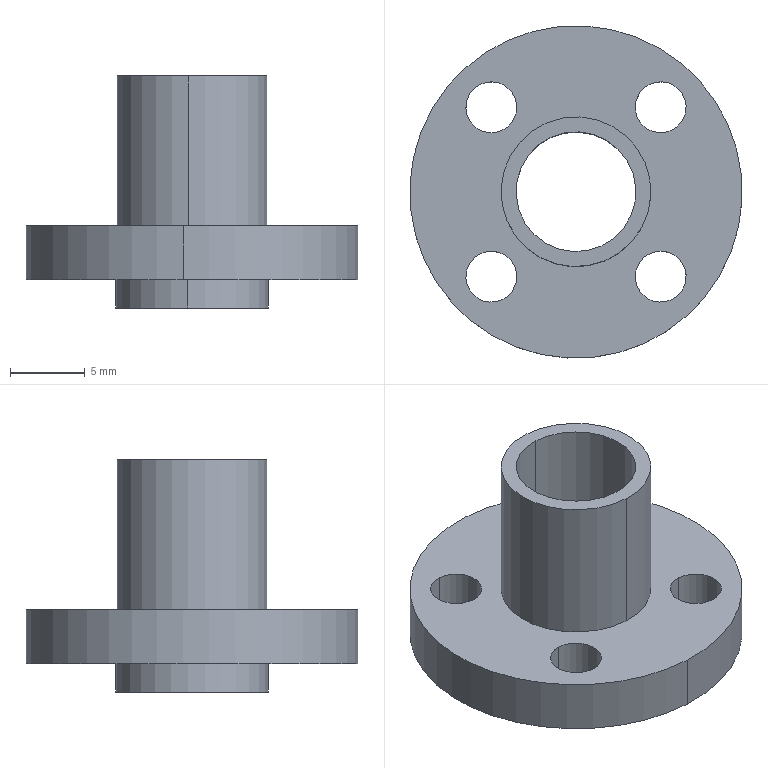Component | SolidWorks | TLeadScrewNut-1 | 1 solid | 20 faces | box 22.2 x 22.2 x 15.5 mm | volume 1424 mm3 | cylinder 16 | plane 4 | commonest cylinder face diameters 3.4 x8 22.2 x2 10 x2 10.2 x2 8 x2
STEP:
#1=COLOUR_RGB('',0.7922,0.8196,0.9333);
#2=FILL_AREA_STYLE_COLOUR('',#1);
#3=FILL_AREA_STYLE('',(#2));
#4=SURFACE_STYLE_FILL_AREA(#3);
#5=SURFACE_SIDE_STYLE('',(#4));
#6=SURFACE_STYLE_USAGE(.BOTH.,#5);
#7=PRESENTATION_STYLE_ASSIGNMENT((#6));
#8=CARTESIAN_POINT('',(-0.02312,-0.4364,2.725));
#9=VERTEX_POINT('',#8);
#10=CARTESIAN_POINT('',(0.02312,0.4364,2.725));
#11=VERTEX_POINT('',#10);
#12=CARTESIAN_POINT('',(-0.,0.,2.725));
#13=DIRECTION('',(-0.,0.,1.));
#14=DIRECTION('',(0.0529,0.9986,0.));
#15=AXIS2_PLACEMENT_3D('',#12,#13,#14);
#16=CIRCLE('',#15,0.437);
#17=EDGE_CURVE('',#9,#11,#16,.T.);
#18=ORIENTED_EDGE('',*,*,#17,.F.);
#19=CARTESIAN_POINT('',(-0.02312,-0.4364,2.583));
#20=VERTEX_POINT('',#19);
#21=CARTESIAN_POINT('',(-0.02312,-0.4364,2.508));
#22=DIRECTION('',(0.,-0.,-1.));
#23=VECTOR('',#22,39.37);
#24=LINE('',#21,#23);
#25=EDGE_CURVE('',#9,#20,#24,.T.);
#26=ORIENTED_EDGE('',*,*,#25,.T.);
#27=CARTESIAN_POINT('',(0.02312,0.4364,2.583));
#28=VERTEX_POINT('',#27);
#29=CARTESIAN_POINT('',(-0.,0.,2.583));
#30=DIRECTION('',(-0.,0.,1.));
#31=DIRECTION('',(0.0529,0.9986,0.));
#32=AXIS2_PLACEMENT_3D('',#29,#30,#31);
#33=CIRCLE('',#32,0.437);
#34=EDGE_CURVE('',#20,#28,#33,.T.);
#35=ORIENTED_EDGE('',*,*,#34,.T.);
#36=CARTESIAN_POINT('',(0.02312,0.4364,2.508));
#37=DIRECTION('',(0.,-0.,-1.));
#38=VECTOR('',#37,39.37);
#39=LINE('',#36,#38);
#40=EDGE_CURVE('',#11,#28,#39,.T.);
#41=ORIENTED_EDGE('',*,*,#40,.F.);
#42=EDGE_LOOP('',(#18,#26,#35,#41));
#43=FACE_OUTER_BOUND('',#42,.T.);
#44=CARTESIAN_POINT('',(-0.,0.,2.508));
#45=DIRECTION('',(0.,-0.,-1.));
#46=DIRECTION('',(0.0529,0.9986,0.));
#47=AXIS2_PLACEMENT_3D('',#44,#45,#46);
#48=CYLINDRICAL_SURFACE('',#47,0.437);
#49=ADVANCED_FACE('',(#43),#48,.T.);
#50=CARTESIAN_POINT('',(0.01041,0.1966,3.119));
#51=VERTEX_POINT('',#50);
#52=CARTESIAN_POINT('',(-0.01041,-0.1966,3.119));
#53=VERTEX_POINT('',#52);
#54=CARTESIAN_POINT('',(-0.,0.,3.119));
#55=DIRECTION('',(0.,-0.,-1.));
#56=DIRECTION('',(0.0529,0.9986,0.));
#57=AXIS2_PLACEMENT_3D('',#54,#55,#56);
#58=CIRCLE('',#57,0.1969);
#59=EDGE_CURVE('',#51,#53,#58,.T.);
#60=ORIENTED_EDGE('',*,*,#59,.T.);
#61=CARTESIAN_POINT('',(-0.01041,-0.1966,2.725));
#62=VERTEX_POINT('',#61);
#63=CARTESIAN_POINT('',(-0.01041,-0.1966,2.508));
#64=DIRECTION('',(0.,-0.,-1.));
#65=VECTOR('',#64,39.37);
#66=LINE('',#63,#65);
#67=EDGE_CURVE('',#53,#62,#66,.T.);
#68=ORIENTED_EDGE('',*,*,#67,.T.);
#69=CARTESIAN_POINT('',(0.01041,0.1966,2.725));
#70=VERTEX_POINT('',#69);
#71=CARTESIAN_POINT('',(-0.,0.,2.725));
#72=DIRECTION('',(0.,-0.,-1.));
#73=DIRECTION('',(0.0529,0.9986,0.));
#74=AXIS2_PLACEMENT_3D('',#71,#72,#73);
#75=CIRCLE('',#74,0.1969);
#76=EDGE_CURVE('',#70,#62,#75,.T.);
#77=ORIENTED_EDGE('',*,*,#76,.F.);
#78=CARTESIAN_POINT('',(0.01041,0.1966,2.508));
#79=DIRECTION('',(0.,-0.,-1.));
#80=VECTOR('',#79,39.37);
#81=LINE('',#78,#80);
#82=EDGE_CURVE('',#51,#70,#81,.T.);
#83=ORIENTED_EDGE('',*,*,#82,.F.);
#84=EDGE_LOOP('',(#60,#68,#77,#83));
#85=FACE_OUTER_BOUND('',#84,.T.);
#86=CARTESIAN_POINT('',(-0.,0.,2.508));
#87=DIRECTION('',(0.,-0.,-1.));
#88=DIRECTION('',(0.0529,0.9986,0.));
#89=AXIS2_PLACEMENT_3D('',#86,#87,#88);
#90=CYLINDRICAL_SURFACE('',#89,0.1969);
#91=ADVANCED_FACE('',(#85),#90,.T.);
#92=CARTESIAN_POINT('',(0.2192,-0.2895,2.725));
#93=VERTEX_POINT('',#92);
#94=CARTESIAN_POINT('',(0.2263,-0.1559,2.725));
#95=VERTEX_POINT('',#94);
#96=CARTESIAN_POINT('',(0.2227,-0.2227,2.725));
#97=DIRECTION('',(0.,-0.,-1.));
#98=DIRECTION('',(0.0529,0.9986,0.));
#99=AXIS2_PLACEMENT_3D('',#96,#97,#98);
#100=CIRCLE('',#99,0.06693);
#101=EDGE_CURVE('',#93,#95,#100,.T.);
#102=ORIENTED_EDGE('',*,*,#101,.F.);
#103=CARTESIAN_POINT('',(0.2192,-0.2895,2.583));
#104=VERTEX_POINT('',#103);
#105=CARTESIAN_POINT('',(0.2192,-0.2895,2.583));
#106=DIRECTION('',(0.,-0.,-1.));
#107=VECTOR('',#106,39.37);
#108=LINE('',#105,#107);
#109=EDGE_CURVE('',#93,#104,#108,.T.);
#110=ORIENTED_EDGE('',*,*,#109,.T.);
#111=CARTESIAN_POINT('',(0.2263,-0.1559,2.583));
#112=VERTEX_POINT('',#111);
#113=CARTESIAN_POINT('',(0.2227,-0.2227,2.583));
#114=DIRECTION('',(-0.,0.,1.));
#115=DIRECTION('',(0.0529,0.9986,0.));
#116=AXIS2_PLACEMENT_3D('',#113,#114,#115);
#117=CIRCLE('',#116,0.06693);
#118=EDGE_CURVE('',#112,#104,#117,.T.);
#119=ORIENTED_EDGE('',*,*,#118,.F.);
#120=CARTESIAN_POINT('',(0.2263,-0.1559,2.583));
#121=DIRECTION('',(0.,-0.,-1.));
#122=VECTOR('',#121,39.37);
#123=LINE('',#120,#122);
#124=EDGE_CURVE('',#95,#112,#123,.T.);
#125=ORIENTED_EDGE('',*,*,#124,.F.);
#126=EDGE_LOOP('',(#102,#110,#119,#125));
#127=FACE_OUTER_BOUND('',#126,.T.);
#128=CARTESIAN_POINT('',(0.2227,-0.2227,2.583));
#129=DIRECTION('',(0.,-0.,-1.));
#130=DIRECTION('',(0.0529,0.9986,0.));
#131=AXIS2_PLACEMENT_3D('',#128,#129,#130);
#132=CYLINDRICAL_SURFACE('',#131,0.06693);
#133=ADVANCED_FACE('',(#127),#132,.F.);
#134=CARTESIAN_POINT('',(-0.2263,-0.2895,2.725));
#135=VERTEX_POINT('',#134);
#136=CARTESIAN_POINT('',(-0.2192,-0.1559,2.725));
#137=VERTEX_POINT('',#136);
#138=CARTESIAN_POINT('',(-0.2227,-0.2227,2.725));
#139=DIRECTION('',(0.,-0.,-1.));
#140=DIRECTION('',(0.0529,0.9986,0.));
#141=AXIS2_PLACEMENT_3D('',#138,#139,#140);
#142=CIRCLE('',#141,0.06693);
#143=EDGE_CURVE('',#135,#137,#142,.T.);
#144=ORIENTED_EDGE('',*,*,#143,.F.);
#145=CARTESIAN_POINT('',(-0.2263,-0.2895,2.583));
#146=VERTEX_POINT('',#145);
#147=CARTESIAN_POINT('',(-0.2263,-0.2895,2.583));
#148=DIRECTION('',(0.,-0.,-1.));
#149=VECTOR('',#148,39.37);
#150=LINE('',#147,#149);
#151=EDGE_CURVE('',#135,#146,#150,.T.);
#152=ORIENTED_EDGE('',*,*,#151,.T.);
#153=CARTESIAN_POINT('',(-0.2192,-0.1559,2.583));
#154=VERTEX_POINT('',#153);
#155=CARTESIAN_POINT('',(-0.2227,-0.2227,2.583));
#156=DIRECTION('',(-0.,0.,1.));
#157=DIRECTION('',(0.0529,0.9986,0.));
#158=AXIS2_PLACEMENT_3D('',#155,#156,#157);
#159=CIRCLE('',#158,0.06693);
#160=EDGE_CURVE('',#154,#146,#159,.T.);
#161=ORIENTED_EDGE('',*,*,#160,.F.);
#162=CARTESIAN_POINT('',(-0.2192,-0.1559,2.583));
#163=DIRECTION('',(0.,-0.,-1.));
#164=VECTOR('',#163,39.37);
#165=LINE('',#162,#164);
#166=EDGE_CURVE('',#137,#154,#165,.T.);
#167=ORIENTED_EDGE('',*,*,#166,.F.);
#168=EDGE_LOOP('',(#144,#152,#161,#167));
#169=FACE_OUTER_BOUND('',#168,.T.);
#170=CARTESIAN_POINT('',(-0.2227,-0.2227,2.583));
#171=DIRECTION('',(0.,-0.,-1.));
#172=DIRECTION('',(0.0529,0.9986,0.));
#173=AXIS2_PLACEMENT_3D('',#170,#171,#172);
#174=CYLINDRICAL_SURFACE('',#173,0.06693);
#175=ADVANCED_FACE('',(#169),#174,.F.);
#176=CARTESIAN_POINT('',(-0.2263,0.1559,2.725));
#177=VERTEX_POINT('',#176);
#178=CARTESIAN_POINT('',(-0.2192,0.2895,2.725));
#179=VERTEX_POINT('',#178);
#180=CARTESIAN_POINT('',(-0.2227,0.2227,2.725));
#181=DIRECTION('',(0.,-0.,-1.));
#182=DIRECTION('',(0.0529,0.9986,0.));
#183=AXIS2_PLACEMENT_3D('',#180,#181,#182);
#184=CIRCLE('',#183,0.06693);
#185=EDGE_CURVE('',#177,#179,#184,.T.);
#186=ORIENTED_EDGE('',*,*,#185,.F.);
#187=CARTESIAN_POINT('',(-0.2263,0.1559,2.583));
#188=VERTEX_POINT('',#187);
#189=CARTESIAN_POINT('',(-0.2263,0.1559,2.583));
#190=DIRECTION('',(0.,-0.,-1.));
#191=VECTOR('',#190,39.37);
#192=LINE('',#189,#191);
#193=EDGE_CURVE('',#177,#188,#192,.T.);
#194=ORIENTED_EDGE('',*,*,#193,.T.);
#195=CARTESIAN_POINT('',(-0.2192,0.2895,2.583));
#196=VERTEX_POINT('',#195);
#197=CARTESIAN_POINT('',(-0.2227,0.2227,2.583));
#198=DIRECTION('',(-0.,0.,1.));
#199=DIRECTION('',(0.0529,0.9986,0.));
#200=AXIS2_PLACEMENT_3D('',#197,#198,#199);
#201=CIRCLE('',#200,0.06693);
#202=EDGE_CURVE('',#196,#188,#201,.T.);
#203=ORIENTED_EDGE('',*,*,#202,.F.);
#204=CARTESIAN_POINT('',(-0.2192,0.2895,2.583));
#205=DIRECTION('',(0.,-0.,-1.));
#206=VECTOR('',#205,39.37);
#207=LINE('',#204,#206);
#208=EDGE_CURVE('',#179,#196,#207,.T.);
#209=ORIENTED_EDGE('',*,*,#208,.F.);
#210=EDGE_LOOP('',(#186,#194,#203,#209));
#211=FACE_OUTER_BOUND('',#210,.T.);
#212=CARTESIAN_POINT('',(-0.2227,0.2227,2.583));
#213=DIRECTION('',(0.,-0.,-1.));
#214=DIRECTION('',(0.0529,0.9986,0.));
#215=AXIS2_PLACEMENT_3D('',#212,#213,#214);
#216=CYLINDRICAL_SURFACE('',#215,0.06693);
#217=ADVANCED_FACE('',(#211),#216,.F.);
#218=CARTESIAN_POINT('',(0.2192,0.1559,2.725));
#219=VERTEX_POINT('',#218);
#220=CARTESIAN_POINT('',(0.2263,0.2895,2.725));
#221=VERTEX_POINT('',#220);
#222=CARTESIAN_POINT('',(0.2227,0.2227,2.725));
#223=DIRECTION('',(0.,-0.,-1.));
#224=DIRECTION('',(0.0529,0.9986,0.));
#225=AXIS2_PLACEMENT_3D('',#222,#223,#224);
#226=CIRCLE('',#225,0.06693);
#227=EDGE_CURVE('',#219,#221,#226,.T.);
#228=ORIENTED_EDGE('',*,*,#227,.F.);
#229=CARTESIAN_POINT('',(0.2192,0.1559,2.583));
#230=VERTEX_POINT('',#229);
#231=CARTESIAN_POINT('',(0.2192,0.1559,2.583));
#232=DIRECTION('',(0.,-0.,-1.));
#233=VECTOR('',#232,39.37);
#234=LINE('',#231,#233);
#235=EDGE_CURVE('',#219,#230,#234,.T.);
#236=ORIENTED_EDGE('',*,*,#235,.T.);
#237=CARTESIAN_POINT('',(0.2263,0.2895,2.583));
#238=VERTEX_POINT('',#237);
#239=CARTESIAN_POINT('',(0.2227,0.2227,2.583));
#240=DIRECTION('',(-0.,0.,1.));
#241=DIRECTION('',(0.0529,0.9986,0.));
#242=AXIS2_PLACEMENT_3D('',#239,#240,#241);
#243=CIRCLE('',#242,0.06693);
#244=EDGE_CURVE('',#238,#230,#243,.T.);
#245=ORIENTED_EDGE('',*,*,#244,.F.);
#246=CARTESIAN_POINT('',(0.2263,0.2895,2.583));
#247=DIRECTION('',(0.,-0.,-1.));
#248=VECTOR('',#247,39.37);
#249=LINE('',#246,#248);
#250=EDGE_CURVE('',#221,#238,#249,.T.);
#251=ORIENTED_EDGE('',*,*,#250,.F.);
#252=EDGE_LOOP('',(#228,#236,#245,#251));
#253=FACE_OUTER_BOUND('',#252,.T.);
#254=CARTESIAN_POINT('',(0.2227,0.2227,2.583));
#255=DIRECTION('',(0.,-0.,-1.));
#256=DIRECTION('',(0.0529,0.9986,0.));
#257=AXIS2_PLACEMENT_3D('',#254,#255,#256);
#258=CYLINDRICAL_SURFACE('',#257,0.06693);
#259=ADVANCED_FACE('',(#253),#258,.F.);
#260=CARTESIAN_POINT('',(-0.01062,-0.2005,2.583));
#261=VERTEX_POINT('',#260);
#262=CARTESIAN_POINT('',(0.01062,0.2005,2.583));
#263=VERTEX_POINT('',#262);
#264=CARTESIAN_POINT('',(-0.,0.,2.583));
#265=DIRECTION('',(-0.,0.,1.));
#266=DIRECTION('',(0.0529,0.9986,0.));
#267=AXIS2_PLACEMENT_3D('',#264,#265,#266);
#268=CIRCLE('',#267,0.2008);
#269=EDGE_CURVE('',#261,#263,#268,.T.);
#270=ORIENTED_EDGE('',*,*,#269,.F.);
#271=CARTESIAN_POINT('',(-0.01062,-0.2005,2.508));
#272=VERTEX_POINT('',#271);
#273=CARTESIAN_POINT('',(-0.01062,-0.2005,2.508));
#274=DIRECTION('',(0.,-0.,-1.));
#275=VECTOR('',#274,39.37);
#276=LINE('',#273,#275);
#277=EDGE_CURVE('',#261,#272,#276,.T.);
#278=ORIENTED_EDGE('',*,*,#277,.T.);
#279=CARTESIAN_POINT('',(0.01062,0.2005,2.508));
#280=VERTEX_POINT('',#279);
#281=CARTESIAN_POINT('',(-0.,0.,2.508));
#282=DIRECTION('',(-0.,0.,1.));
#283=DIRECTION('',(0.0529,0.9986,0.));
#284=AXIS2_PLACEMENT_3D('',#281,#282,#283);
#285=CIRCLE('',#284,0.2008);
#286=EDGE_CURVE('',#272,#280,#285,.T.);
#287=ORIENTED_EDGE('',*,*,#286,.T.);
#288=CARTESIAN_POINT('',(0.01062,0.2005,2.508));
#289=DIRECTION('',(0.,-0.,-1.));
#290=VECTOR('',#289,39.37);
#291=LINE('',#288,#290);
#292=EDGE_CURVE('',#263,#280,#291,.T.);
#293=ORIENTED_EDGE('',*,*,#292,.F.);
#294=EDGE_LOOP('',(#270,#278,#287,#293));
#295=FACE_OUTER_BOUND('',#294,.T.);
#296=CARTESIAN_POINT('',(-0.,0.,2.508));
#297=DIRECTION('',(0.,-0.,-1.));
#298=DIRECTION('',(0.0529,0.9986,0.));
#299=AXIS2_PLACEMENT_3D('',#296,#297,#298);
#300=CYLINDRICAL_SURFACE('',#299,0.2008);
#301=ADVANCED_FACE('',(#295),#300,.T.);
#302=CARTESIAN_POINT('',(-0.00833,-0.1573,3.119));
#303=VERTEX_POINT('',#302);
#304=CARTESIAN_POINT('',(0.00833,0.1573,3.119));
#305=VERTEX_POINT('',#304);
#306=CARTESIAN_POINT('',(-0.,0.,3.119));
#307=DIRECTION('',(0.,-0.,-1.));
#308=DIRECTION('',(0.0529,0.9986,0.));
#309=AXIS2_PLACEMENT_3D('',#306,#307,#308);
#310=CIRCLE('',#309,0.1575);
#311=EDGE_CURVE('',#303,#305,#310,.T.);
#312=ORIENTED_EDGE('',*,*,#311,.F.);
#313=CARTESIAN_POINT('',(-0.00833,-0.1573,2.508));
#314=VERTEX_POINT('',#313);
#315=CARTESIAN_POINT('',(-0.00833,-0.1573,2.508));
#316=DIRECTION('',(0.,-0.,-1.));
#317=VECTOR('',#316,39.37);
#318=LINE('',#315,#317);
#319=EDGE_CURVE('',#303,#314,#318,.T.);
#320=ORIENTED_EDGE('',*,*,#319,.T.);
#321=CARTESIAN_POINT('',(0.00833,0.1573,2.508));
#322=VERTEX_POINT('',#321);
#323=CARTESIAN_POINT('',(-0.,0.,2.508));
#324=DIRECTION('',(-0.,0.,1.));
#325=DIRECTION('',(0.0529,0.9986,0.));
#326=AXIS2_PLACEMENT_3D('',#323,#324,#325);
#327=CIRCLE('',#326,0.1575);
#328=EDGE_CURVE('',#322,#314,#327,.T.);
#329=ORIENTED_EDGE('',*,*,#328,.F.);
#330=CARTESIAN_POINT('',(0.00833,0.1573,2.508));
#331=DIRECTION('',(0.,-0.,-1.));
#332=VECTOR('',#331,39.37);
#333=LINE('',#330,#332);
#334=EDGE_CURVE('',#305,#322,#333,.T.);
#335=ORIENTED_EDGE('',*,*,#334,.F.);
#336=EDGE_LOOP('',(#312,#320,#329,#335));
#337=FACE_OUTER_BOUND('',#336,.T.);
#338=CARTESIAN_POINT('',(-0.,0.,2.508));
#339=DIRECTION('',(0.,-0.,-1.));
#340=DIRECTION('',(0.0529,0.9986,0.));
#341=AXIS2_PLACEMENT_3D('',#338,#339,#340);
#342=CYLINDRICAL_SURFACE('',#341,0.1575);
#343=ADVANCED_FACE('',(#337),#342,.F.);
#344=CARTESIAN_POINT('',(-0.,0.,2.725));
#345=DIRECTION('',(-0.,0.,1.));
#346=DIRECTION('',(0.0529,0.9986,0.));
#347=AXIS2_PLACEMENT_3D('',#344,#345,#346);
#348=CIRCLE('',#347,0.437);
#349=EDGE_CURVE('',#11,#9,#348,.T.);
#350=ORIENTED_EDGE('',*,*,#349,.T.);
#351=ORIENTED_EDGE('',*,*,#17,.T.);
#352=EDGE_LOOP('',(#350,#351));
#353=FACE_OUTER_BOUND('',#352,.T.);
#354=ORIENTED_EDGE('',*,*,#76,.T.);
#355=CARTESIAN_POINT('',(-0.,0.,2.725));
#356=DIRECTION('',(0.,-0.,-1.));
#357=DIRECTION('',(0.0529,0.9986,0.));
#358=AXIS2_PLACEMENT_3D('',#355,#356,#357);
#359=CIRCLE('',#358,0.1969);
#360=EDGE_CURVE('',#62,#70,#359,.T.);
#361=ORIENTED_EDGE('',*,*,#360,.T.);
#362=EDGE_LOOP('',(#354,#361));
#363=FACE_BOUND('',#362,.T.);
#364=CARTESIAN_POINT('',(0.2227,-0.2227,2.725));
#365=DIRECTION('',(0.,-0.,-1.));
#366=DIRECTION('',(0.0529,0.9986,0.));
#367=AXIS2_PLACEMENT_3D('',#364,#365,#366);
#368=CIRCLE('',#367,0.06693);
#369=EDGE_CURVE('',#95,#93,#368,.T.);
#370=ORIENTED_EDGE('',*,*,#369,.T.);
#371=ORIENTED_EDGE('',*,*,#101,.T.);
#372=EDGE_LOOP('',(#370,#371));
#373=FACE_BOUND('',#372,.T.);
#374=CARTESIAN_POINT('',(-0.2227,-0.2227,2.725));
#375=DIRECTION('',(0.,-0.,-1.));
#376=DIRECTION('',(0.0529,0.9986,0.));
#377=AXIS2_PLACEMENT_3D('',#374,#375,#376);
#378=CIRCLE('',#377,0.06693);
#379=EDGE_CURVE('',#137,#135,#378,.T.);
#380=ORIENTED_EDGE('',*,*,#379,.T.);
#381=ORIENTED_EDGE('',*,*,#143,.T.);
#382=EDGE_LOOP('',(#380,#381));
#383=FACE_BOUND('',#382,.T.);
#384=CARTESIAN_POINT('',(-0.2227,0.2227,2.725));
#385=DIRECTION('',(0.,-0.,-1.));
#386=DIRECTION('',(0.0529,0.9986,0.));
#387=AXIS2_PLACEMENT_3D('',#384,#385,#386);
#388=CIRCLE('',#387,0.06693);
#389=EDGE_CURVE('',#179,#177,#388,.T.);
#390=ORIENTED_EDGE('',*,*,#389,.T.);
#391=ORIENTED_EDGE('',*,*,#185,.T.);
#392=EDGE_LOOP('',(#390,#391));
#393=FACE_BOUND('',#392,.T.);
#394=CARTESIAN_POINT('',(0.2227,0.2227,2.725));
#395=DIRECTION('',(0.,-0.,-1.));
#396=DIRECTION('',(0.0529,0.9986,0.));
#397=AXIS2_PLACEMENT_3D('',#394,#395,#396);
#398=CIRCLE('',#397,0.06693);
#399=EDGE_CURVE('',#221,#219,#398,.T.);
#400=ORIENTED_EDGE('',*,*,#399,.T.);
#401=ORIENTED_EDGE('',*,*,#227,.T.);
#402=EDGE_LOOP('',(#400,#401));
#403=FACE_BOUND('',#402,.T.);
#404=CARTESIAN_POINT('',(-0.,0.,2.725));
#405=DIRECTION('',(-0.,0.,1.));
#406=DIRECTION('',(-0.0529,-0.9986,0.));
#407=AXIS2_PLACEMENT_3D('',#404,#405,#406);
#408=PLANE('',#407);
#409=ADVANCED_FACE('',(#353,#363,#373,#383,#393,#403),#408,.T.);
#410=ORIENTED_EDGE('',*,*,#25,.F.);
#411=ORIENTED_EDGE('',*,*,#349,.F.);
#412=ORIENTED_EDGE('',*,*,#40,.T.);
#413=CARTESIAN_POINT('',(-0.,0.,2.583));
#414=DIRECTION('',(-0.,0.,1.));
#415=DIRECTION('',(0.0529,0.9986,0.));
#416=AXIS2_PLACEMENT_3D('',#413,#414,#415);
#417=CIRCLE('',#416,0.437);
#418=EDGE_CURVE('',#28,#20,#417,.T.);
#419=ORIENTED_EDGE('',*,*,#418,.T.);
#420=EDGE_LOOP('',(#410,#411,#412,#419));
#421=FACE_OUTER_BOUND('',#420,.T.);
#422=CARTESIAN_POINT('',(-0.,0.,2.508));
#423=DIRECTION('',(0.,-0.,-1.));
#424=DIRECTION('',(0.0529,0.9986,0.));
#425=AXIS2_PLACEMENT_3D('',#422,#423,#424);
#426=CYLINDRICAL_SURFACE('',#425,0.437);
#427=ADVANCED_FACE('',(#421),#426,.T.);
#428=ORIENTED_EDGE('',*,*,#67,.F.);
#429=CARTESIAN_POINT('',(-0.,0.,3.119));
#430=DIRECTION('',(0.,-0.,-1.));
#431=DIRECTION('',(0.0529,0.9986,0.));
#432=AXIS2_PLACEMENT_3D('',#429,#430,#431);
#433=CIRCLE('',#432,0.1969);
#434=EDGE_CURVE('',#53,#51,#433,.T.);
#435=ORIENTED_EDGE('',*,*,#434,.T.);
#436=ORIENTED_EDGE('',*,*,#82,.T.);
#437=ORIENTED_EDGE('',*,*,#360,.F.);
#438=EDGE_LOOP('',(#428,#435,#436,#437));
#439=FACE_OUTER_BOUND('',#438,.T.);
#440=CARTESIAN_POINT('',(-0.,0.,2.508));
#441=DIRECTION('',(0.,-0.,-1.));
#442=DIRECTION('',(0.0529,0.9986,0.));
#443=AXIS2_PLACEMENT_3D('',#440,#441,#442);
#444=CYLINDRICAL_SURFACE('',#443,0.1969);
#445=ADVANCED_FACE('',(#439),#444,.T.);
#446=ORIENTED_EDGE('',*,*,#109,.F.);
#447=ORIENTED_EDGE('',*,*,#369,.F.);
#448=ORIENTED_EDGE('',*,*,#124,.T.);
#449=CARTESIAN_POINT('',(0.2227,-0.2227,2.583));
#450=DIRECTION('',(-0.,0.,1.));
#451=DIRECTION('',(0.0529,0.9986,0.));
#452=AXIS2_PLACEMENT_3D('',#449,#450,#451);
#453=CIRCLE('',#452,0.06693);
#454=EDGE_CURVE('',#104,#112,#453,.T.);
#455=ORIENTED_EDGE('',*,*,#454,.F.);
#456=EDGE_LOOP('',(#446,#447,#448,#455));
#457=FACE_OUTER_BOUND('',#456,.T.);
#458=CARTESIAN_POINT('',(0.2227,-0.2227,2.583));
#459=DIRECTION('',(0.,-0.,-1.));
#460=DIRECTION('',(0.0529,0.9986,0.));
#461=AXIS2_PLACEMENT_3D('',#458,#459,#460);
#462=CYLINDRICAL_SURFACE('',#461,0.06693);
#463=ADVANCED_FACE('',(#457),#462,.F.);
#464=ORIENTED_EDGE('',*,*,#151,.F.);
#465=ORIENTED_EDGE('',*,*,#379,.F.);
#466=ORIENTED_EDGE('',*,*,#166,.T.);
#467=CARTESIAN_POINT('',(-0.2227,-0.2227,2.583));
#468=DIRECTION('',(-0.,0.,1.));
#469=DIRECTION('',(0.0529,0.9986,0.));
#470=AXIS2_PLACEMENT_3D('',#467,#468,#469);
#471=CIRCLE('',#470,0.06693);
#472=EDGE_CURVE('',#146,#154,#471,.T.);
#473=ORIENTED_EDGE('',*,*,#472,.F.);
#474=EDGE_LOOP('',(#464,#465,#466,#473));
#475=FACE_OUTER_BOUND('',#474,.T.);
#476=CARTESIAN_POINT('',(-0.2227,-0.2227,2.583));
#477=DIRECTION('',(0.,-0.,-1.));
#478=DIRECTION('',(0.0529,0.9986,0.));
#479=AXIS2_PLACEMENT_3D('',#476,#477,#478);
#480=CYLINDRICAL_SURFACE('',#479,0.06693);
#481=ADVANCED_FACE('',(#475),#480,.F.);
#482=ORIENTED_EDGE('',*,*,#193,.F.);
#483=ORIENTED_EDGE('',*,*,#389,.F.);
#484=ORIENTED_EDGE('',*,*,#208,.T.);
#485=CARTESIAN_POINT('',(-0.2227,0.2227,2.583));
#486=DIRECTION('',(-0.,0.,1.));
#487=DIRECTION('',(0.0529,0.9986,0.));
#488=AXIS2_PLACEMENT_3D('',#485,#486,#487);
#489=CIRCLE('',#488,0.06693);
#490=EDGE_CURVE('',#188,#196,#489,.T.);
#491=ORIENTED_EDGE('',*,*,#490,.F.);
#492=EDGE_LOOP('',(#482,#483,#484,#491));
#493=FACE_OUTER_BOUND('',#492,.T.);
#494=CARTESIAN_POINT('',(-0.2227,0.2227,2.583));
#495=DIRECTION('',(0.,-0.,-1.));
#496=DIRECTION('',(0.0529,0.9986,0.));
#497=AXIS2_PLACEMENT_3D('',#494,#495,#496);
#498=CYLINDRICAL_SURFACE('',#497,0.06693);
#499=ADVANCED_FACE('',(#493),#498,.F.);
#500=ORIENTED_EDGE('',*,*,#235,.F.);
#501=ORIENTED_EDGE('',*,*,#399,.F.);
#502=ORIENTED_EDGE('',*,*,#250,.T.);
#503=CARTESIAN_POINT('',(0.2227,0.2227,2.583));
#504=DIRECTION('',(-0.,0.,1.));
#505=DIRECTION('',(0.0529,0.9986,0.));
#506=AXIS2_PLACEMENT_3D('',#503,#504,#505);
#507=CIRCLE('',#506,0.06693);
#508=EDGE_CURVE('',#230,#238,#507,.T.);
#509=ORIENTED_EDGE('',*,*,#508,.F.);
#510=EDGE_LOOP('',(#500,#501,#502,#509));
#511=FACE_OUTER_BOUND('',#510,.T.);
#512=CARTESIAN_POINT('',(0.2227,0.2227,2.583));
#513=DIRECTION('',(0.,-0.,-1.));
#514=DIRECTION('',(0.0529,0.9986,0.));
#515=AXIS2_PLACEMENT_3D('',#512,#513,#514);
#516=CYLINDRICAL_SURFACE('',#515,0.06693);
#517=ADVANCED_FACE('',(#511),#516,.F.);
#518=CARTESIAN_POINT('',(-0.,0.,2.583));
#519=DIRECTION('',(-0.,0.,1.));
#520=DIRECTION('',(0.0529,0.9986,0.));
#521=AXIS2_PLACEMENT_3D('',#518,#519,#520);
#522=CIRCLE('',#521,0.2008);
#523=EDGE_CURVE('',#263,#261,#522,.T.);
#524=ORIENTED_EDGE('',*,*,#523,.T.);
#525=ORIENTED_EDGE('',*,*,#269,.T.);
#526=EDGE_LOOP('',(#524,#525));
#527=FACE_BOUND('',#526,.T.);
#528=ORIENTED_EDGE('',*,*,#418,.F.);
#529=ORIENTED_EDGE('',*,*,#34,.F.);
#530=EDGE_LOOP('',(#528,#529));
#531=FACE_OUTER_BOUND('',#530,.T.);
#532=ORIENTED_EDGE('',*,*,#118,.T.);
#533=ORIENTED_EDGE('',*,*,#454,.T.);
#534=EDGE_LOOP('',(#532,#533));
#535=FACE_BOUND('',#534,.T.);
#536=ORIENTED_EDGE('',*,*,#160,.T.);
#537=ORIENTED_EDGE('',*,*,#472,.T.);
#538=EDGE_LOOP('',(#536,#537));
#539=FACE_BOUND('',#538,.T.);
#540=ORIENTED_EDGE('',*,*,#202,.T.);
#541=ORIENTED_EDGE('',*,*,#490,.T.);
#542=EDGE_LOOP('',(#540,#541));
#543=FACE_BOUND('',#542,.T.);
#544=ORIENTED_EDGE('',*,*,#244,.T.);
#545=ORIENTED_EDGE('',*,*,#508,.T.);
#546=EDGE_LOOP('',(#544,#545));
#547=FACE_BOUND('',#546,.T.);
#548=CARTESIAN_POINT('',(-0.,0.,2.583));
#549=DIRECTION('',(0.,-0.,-1.));
#550=DIRECTION('',(0.0529,0.9986,-0.));
#551=AXIS2_PLACEMENT_3D('',#548,#549,#550);
#552=PLANE('',#551);
#553=ADVANCED_FACE('',(#527,#531,#535,#539,#543,#547),#552,.T.);
#554=ORIENTED_EDGE('',*,*,#59,.F.);
#555=ORIENTED_EDGE('',*,*,#434,.F.);
#556=EDGE_LOOP('',(#554,#555));
#557=FACE_OUTER_BOUND('',#556,.T.);
#558=CARTESIAN_POINT('',(-0.,0.,3.119));
#559=DIRECTION('',(0.,-0.,-1.));
#560=DIRECTION('',(0.0529,0.9986,0.));
#561=AXIS2_PLACEMENT_3D('',#558,#559,#560);
#562=CIRCLE('',#561,0.1575);
#563=EDGE_CURVE('',#305,#303,#562,.T.);
#564=ORIENTED_EDGE('',*,*,#563,.T.);
#565=ORIENTED_EDGE('',*,*,#311,.T.);
#566=EDGE_LOOP('',(#564,#565));
#567=FACE_BOUND('',#566,.T.);
#568=CARTESIAN_POINT('',(-0.,0.,3.119));
#569=DIRECTION('',(-0.,0.,1.));
#570=DIRECTION('',(-0.0529,-0.9986,0.));
#571=AXIS2_PLACEMENT_3D('',#568,#569,#570);
#572=PLANE('',#571);
#573=ADVANCED_FACE('',(#557,#567),#572,.T.);
#574=ORIENTED_EDGE('',*,*,#277,.F.);
#575=ORIENTED_EDGE('',*,*,#523,.F.);
#576=ORIENTED_EDGE('',*,*,#292,.T.);
#577=CARTESIAN_POINT('',(-0.,0.,2.508));
#578=DIRECTION('',(-0.,0.,1.));
#579=DIRECTION('',(0.0529,0.9986,0.));
#580=AXIS2_PLACEMENT_3D('',#577,#578,#579);
#581=CIRCLE('',#580,0.2008);
#582=EDGE_CURVE('',#280,#272,#581,.T.);
#583=ORIENTED_EDGE('',*,*,#582,.T.);
#584=EDGE_LOOP('',(#574,#575,#576,#583));
#585=FACE_OUTER_BOUND('',#584,.T.);
#586=CARTESIAN_POINT('',(-0.,0.,2.508));
#587=DIRECTION('',(0.,-0.,-1.));
#588=DIRECTION('',(0.0529,0.9986,0.));
#589=AXIS2_PLACEMENT_3D('',#586,#587,#588);
#590=CYLINDRICAL_SURFACE('',#589,0.2008);
#591=ADVANCED_FACE('',(#585),#590,.T.);
#592=ORIENTED_EDGE('',*,*,#319,.F.);
#593=ORIENTED_EDGE('',*,*,#563,.F.);
#594=ORIENTED_EDGE('',*,*,#334,.T.);
#595=CARTESIAN_POINT('',(-0.,0.,2.508));
#596=DIRECTION('',(-0.,0.,1.));
#597=DIRECTION('',(0.0529,0.9986,0.));
#598=AXIS2_PLACEMENT_3D('',#595,#596,#597);
#599=CIRCLE('',#598,0.1575);
#600=EDGE_CURVE('',#314,#322,#599,.T.);
#601=ORIENTED_EDGE('',*,*,#600,.F.);
#602=EDGE_LOOP('',(#592,#593,#594,#601));
#603=FACE_OUTER_BOUND('',#602,.T.);
#604=CARTESIAN_POINT('',(-0.,0.,2.508));
#605=DIRECTION('',(0.,-0.,-1.));
#606=DIRECTION('',(0.0529,0.9986,0.));
#607=AXIS2_PLACEMENT_3D('',#604,#605,#606);
#608=CYLINDRICAL_SURFACE('',#607,0.1575);
#609=ADVANCED_FACE('',(#603),#608,.F.);
#610=ORIENTED_EDGE('',*,*,#328,.T.);
#611=ORIENTED_EDGE('',*,*,#600,.T.);
#612=EDGE_LOOP('',(#610,#611));
#613=FACE_BOUND('',#612,.T.);
#614=ORIENTED_EDGE('',*,*,#582,.F.);
#615=ORIENTED_EDGE('',*,*,#286,.F.);
#616=EDGE_LOOP('',(#614,#615));
#617=FACE_OUTER_BOUND('',#616,.T.);
#618=CARTESIAN_POINT('',(-0.,0.,2.508));
#619=DIRECTION('',(0.,-0.,-1.));
#620=DIRECTION('',(0.0529,0.9986,-0.));
#621=AXIS2_PLACEMENT_3D('',#618,#619,#620);
#622=PLANE('',#621);
#623=ADVANCED_FACE('',(#613,#617),#622,.T.);
#624=CLOSED_SHELL('',(#49,#91,#133,#175,#217,#259,#301,#343,#409,#427,#445,#463,#481,#499,#517,#553,#573,#591,#609,#623));
#625=MANIFOLD_SOLID_BREP('',#624);
#626=STYLED_ITEM('',(#7),#625);
#627=PRESENTATION_LAYER_ASSIGNMENT('','',(#626));
#628=CARTESIAN_POINT('',(0.,0.,0.));
#629=DIRECTION('',(0.,0.,1.));
#630=DIRECTION('',(1.,0.,0.));
#631=AXIS2_PLACEMENT_3D('',#628,#629,#630);
#632=(LENGTH_UNIT()NAMED_UNIT(*)SI_UNIT($,.METRE.));
#633=LENGTH_MEASURE_WITH_UNIT(LENGTH_MEASURE(0.0254),#632);
#634=DIMENSIONAL_EXPONENTS(1.,0.,0.,0.,0.,0.,0.);
#635=(CONVERSION_BASED_UNIT('',#633)LENGTH_UNIT()NAMED_UNIT(#634));
#636=UNCERTAINTY_MEASURE_WITH_UNIT(LENGTH_MEASURE(0.00001),#635,'','');
#637=(NAMED_UNIT(*)PLANE_ANGLE_UNIT()SI_UNIT($,.RADIAN.));
#638=(NAMED_UNIT(*)SI_UNIT($,.STERADIAN.)SOLID_ANGLE_UNIT());
#639=(GEOMETRIC_REPRESENTATION_CONTEXT(3)GLOBAL_UNCERTAINTY_ASSIGNED_CONTEXT((#636))GLOBAL_UNIT_ASSIGNED_CONTEXT((#635,#637,#638))REPRESENTATION_CONTEXT('',''));
#640=ADVANCED_BREP_SHAPE_REPRESENTATION('',(#625,#631),#639);
#641=(LENGTH_UNIT()NAMED_UNIT(*)SI_UNIT($,.METRE.));
#642=LENGTH_MEASURE_WITH_UNIT(LENGTH_MEASURE(0.0254),#641);
#643=DIMENSIONAL_EXPONENTS(1.,0.,0.,0.,0.,0.,0.);
#644=(CONVERSION_BASED_UNIT('',#642)LENGTH_UNIT()NAMED_UNIT(#643));
#645=UNCERTAINTY_MEASURE_WITH_UNIT(LENGTH_MEASURE(0.00001),#644,'','');
#646=(NAMED_UNIT(*)PLANE_ANGLE_UNIT()SI_UNIT($,.RADIAN.));
#647=(NAMED_UNIT(*)SI_UNIT($,.STERADIAN.)SOLID_ANGLE_UNIT());
#648=(GEOMETRIC_REPRESENTATION_CONTEXT(3)GLOBAL_UNCERTAINTY_ASSIGNED_CONTEXT((#645))GLOBAL_UNIT_ASSIGNED_CONTEXT((#644,#646,#647))REPRESENTATION_CONTEXT('',''));
#649=MECHANICAL_DESIGN_GEOMETRIC_PRESENTATION_REPRESENTATION('',(#626),#648);